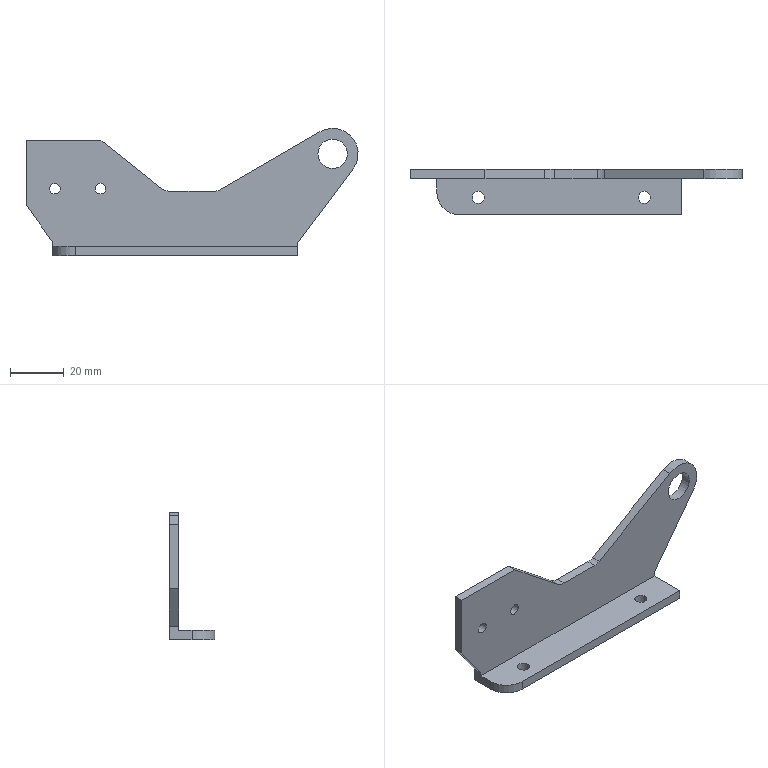Component | NX | SIDE_PLATE | 1 solid | 23 faces | volume 17412 mm3 | plane 14 | cylinder 9 | commonest cylinder face diameters 4 x2 4.5 x2 17 x1 19 x1 10 x1 12 x1 11 x1